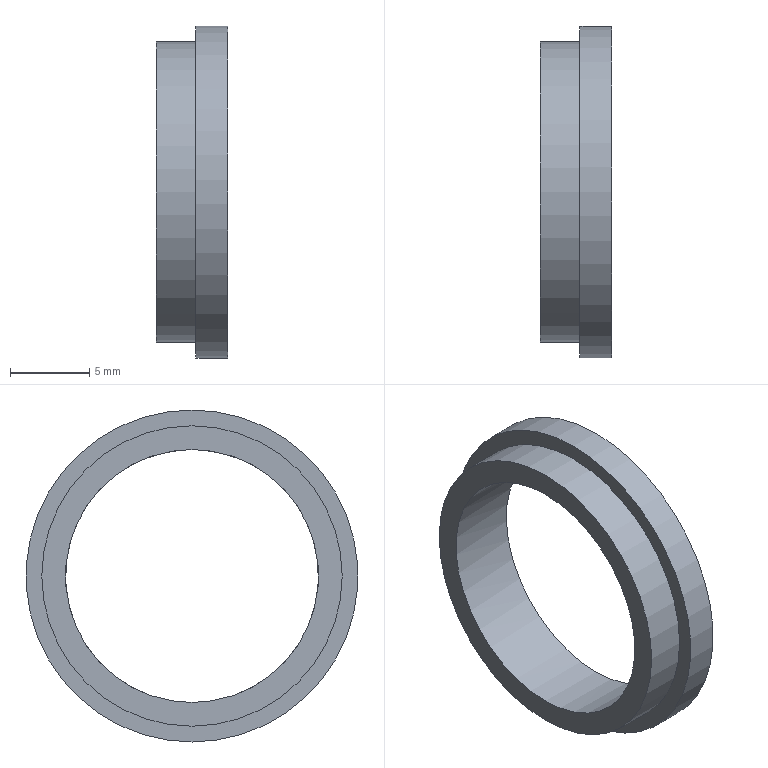Component | NX | END_CAP_4_BUSHING | 1 solid | 6 faces | volume 497 mm3 | plane 3 | cylinder 3 | commonest cylinder face diameters 19 x1 21 x1 16 x1